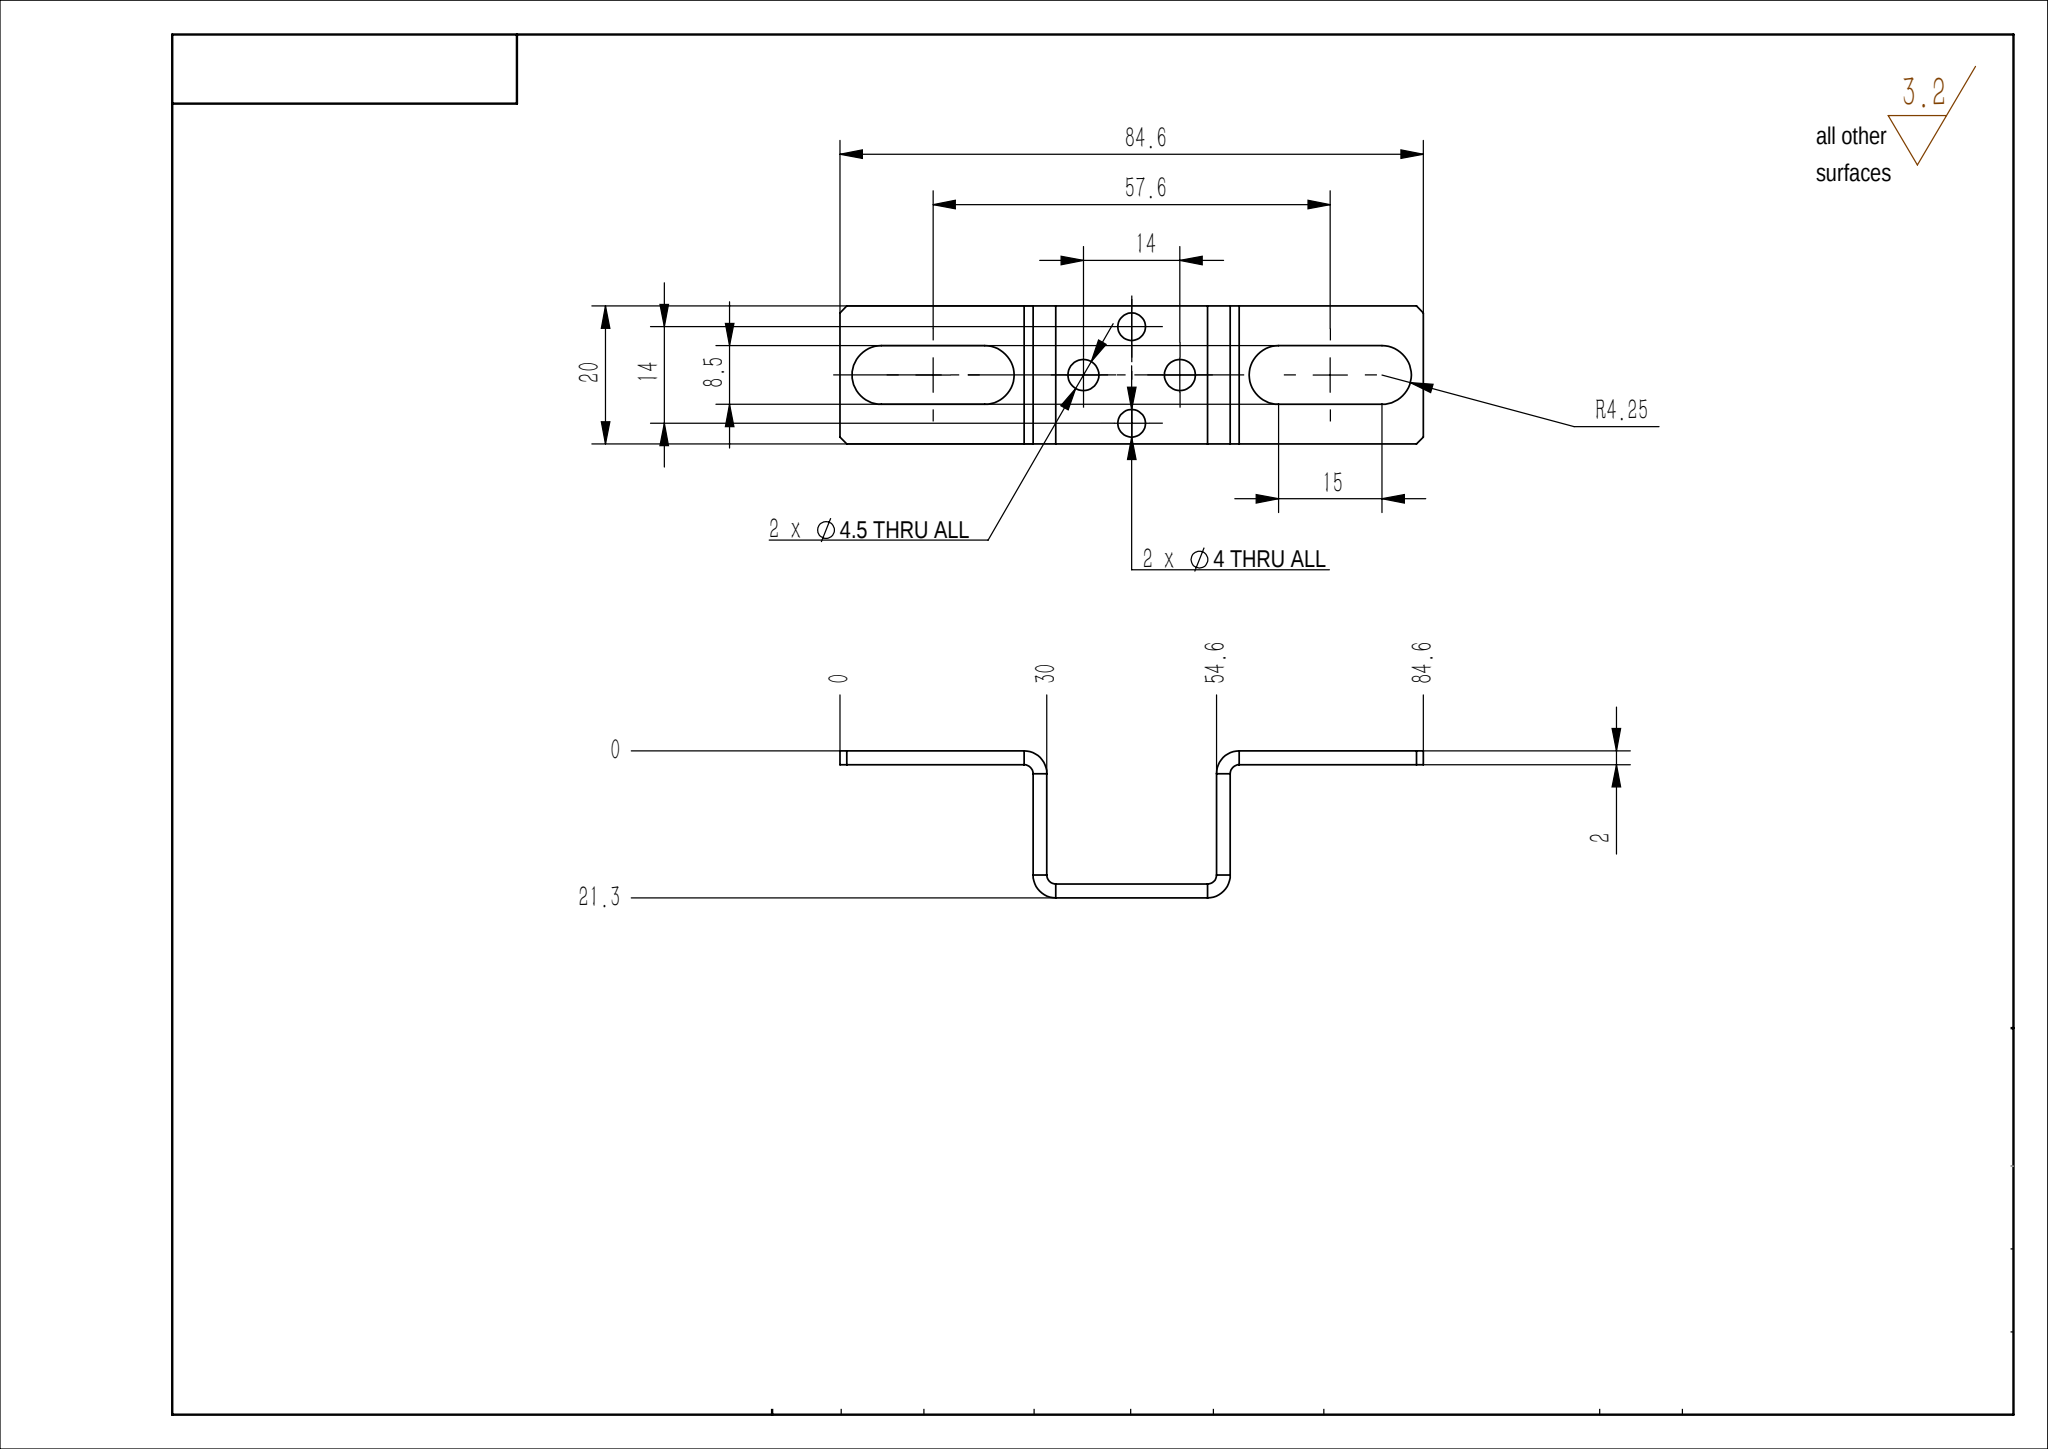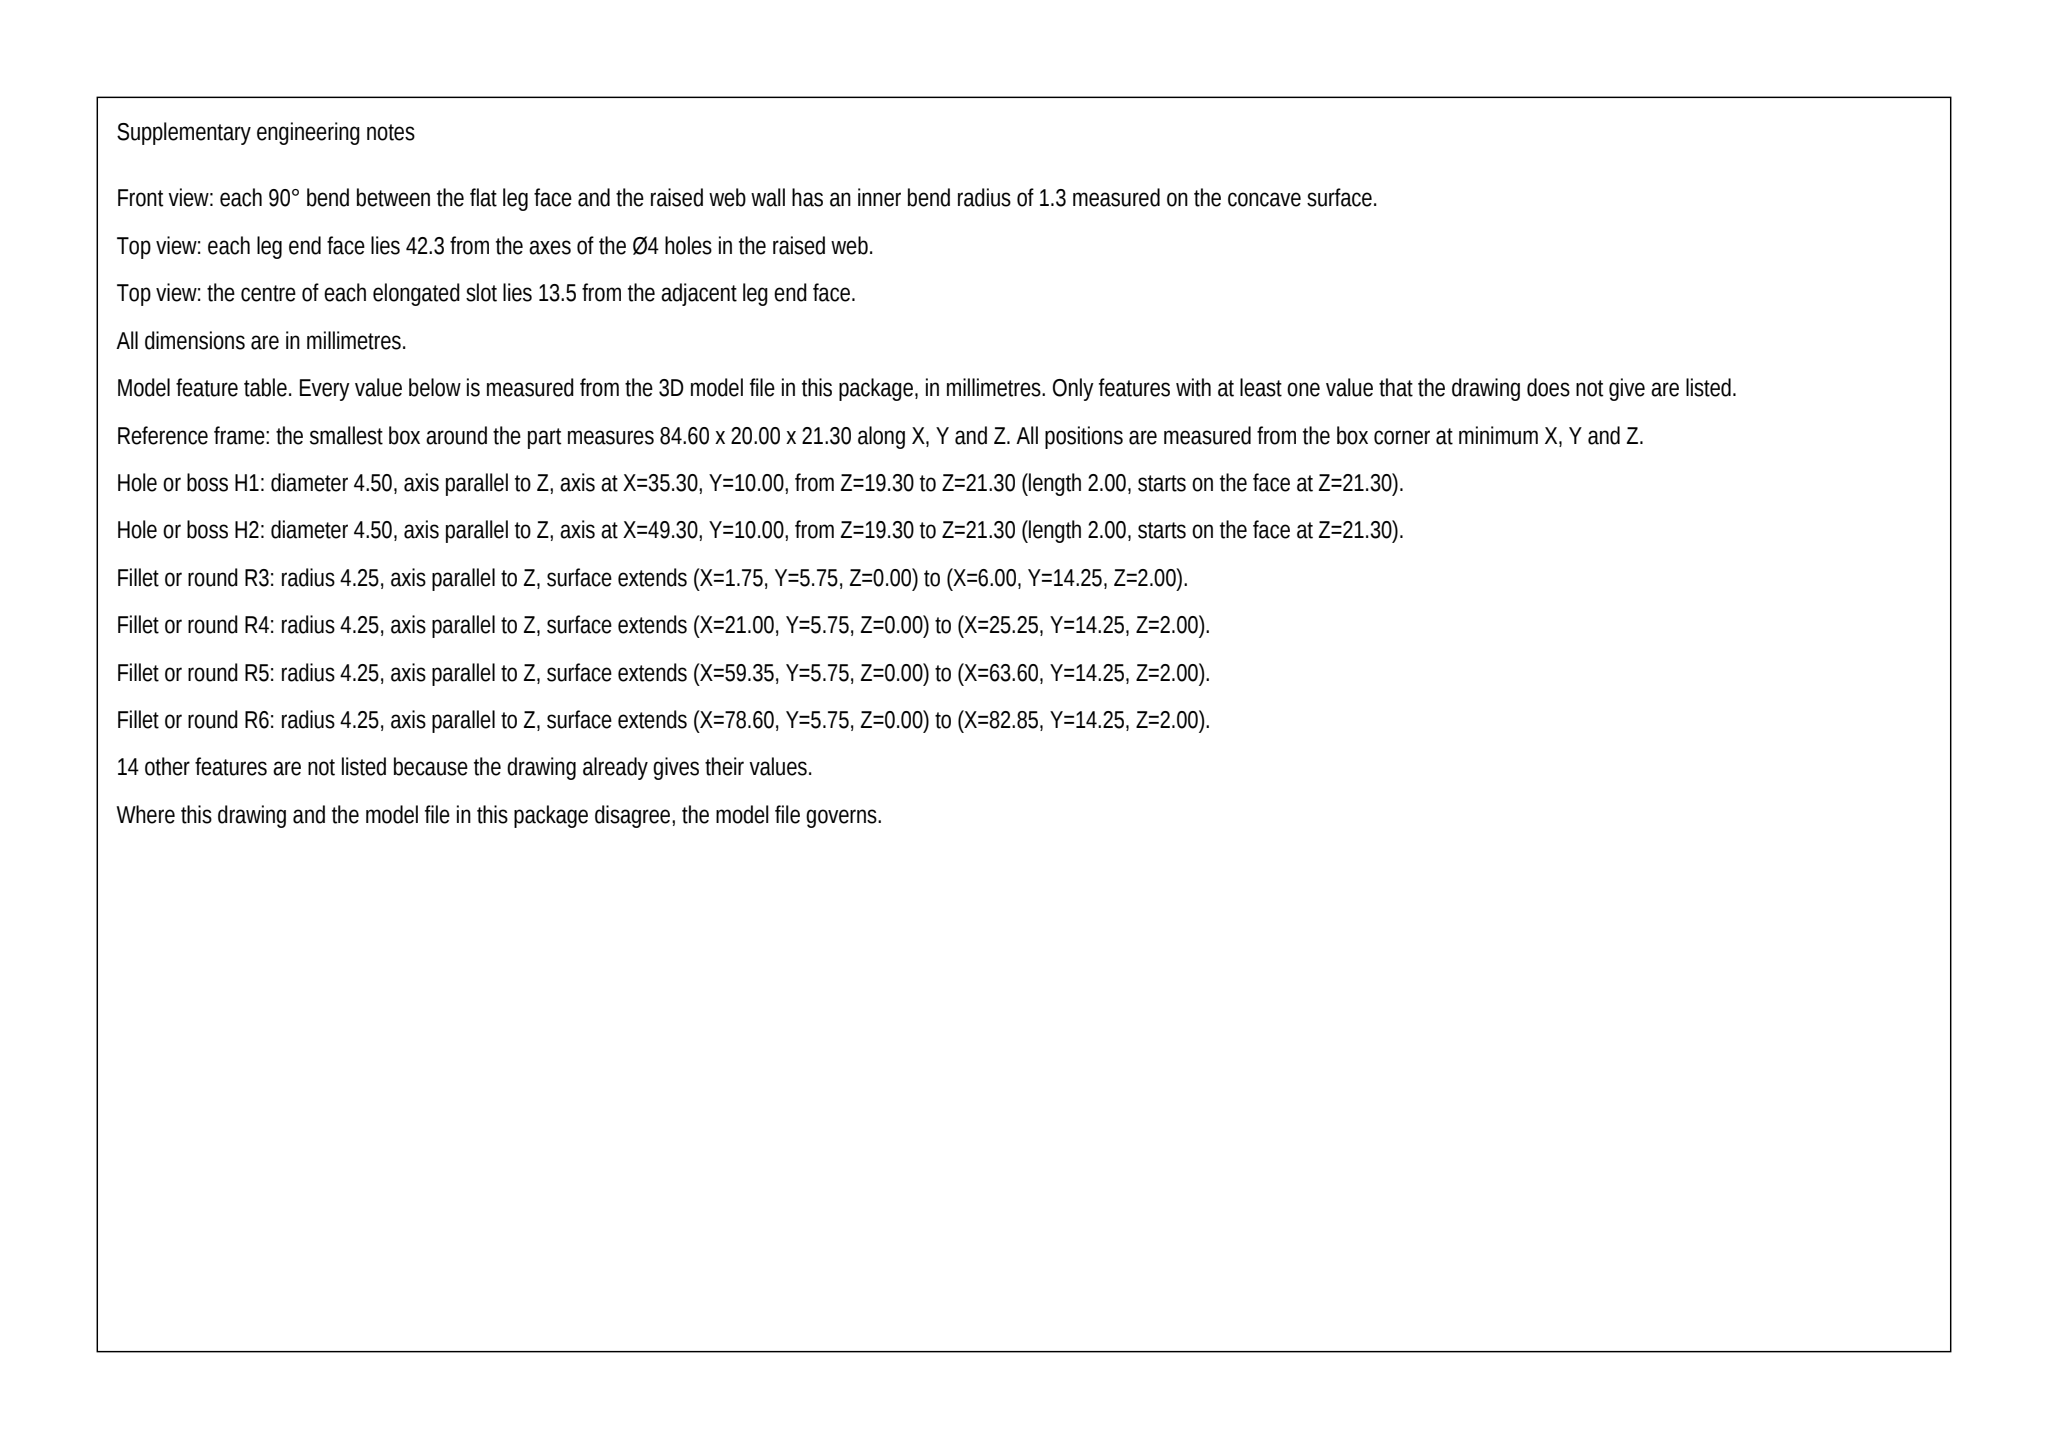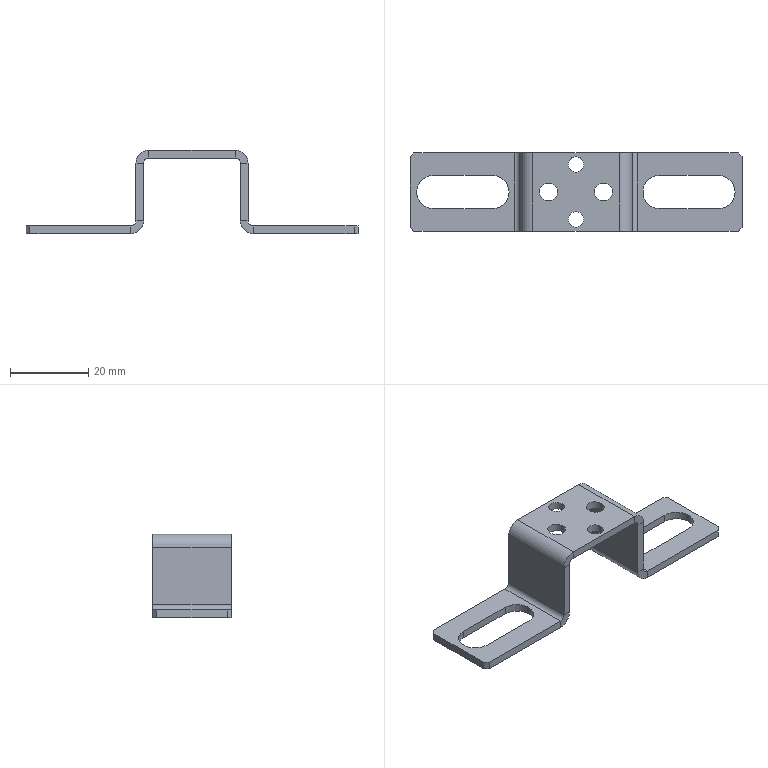Part | SolidWorks | mm | 1 solid | 60 faces | box 84.6 x 20 x 21.3 mm | volume 3915 mm3 | plane 38 | cylinder 22 | commonest cylinder face diameters 8.5 x6 4 x4 4.5 x4 6.6 x4 2.6 x4